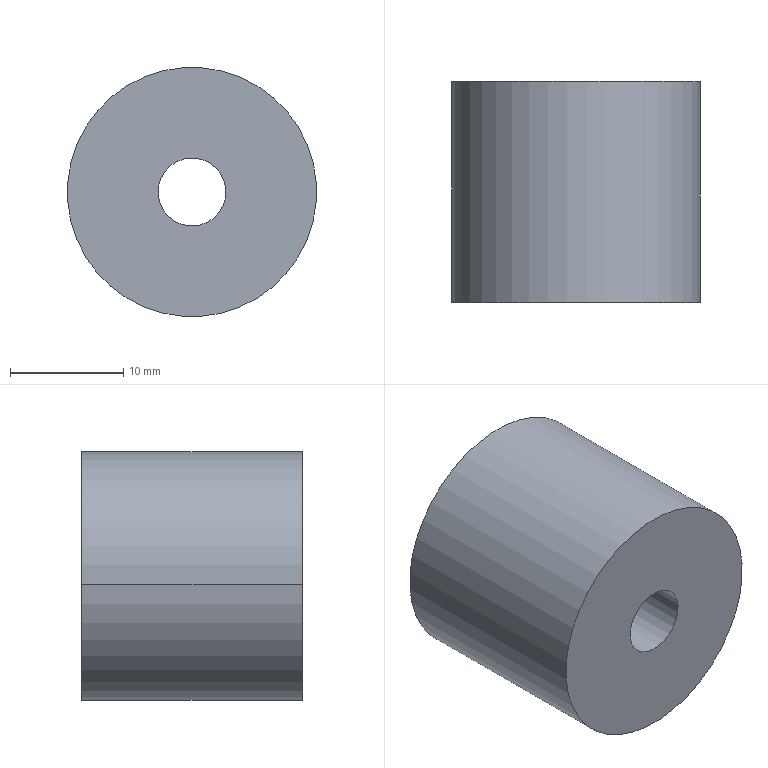Component | SolidWorks | RotaryCylinderSupportPost-1 | 1 solid | 6 faces | box 22 x 19.5 x 22 mm | volume 6861 mm3 | cylinder 4 | plane 2 | commonest cylinder face diameters 6 x2 22 x2
build123d program:
from build123d import *

# Parameters (mm, degrees)
SKETCH2_R           = 11
SKETCH2_R_2         = 3
BOSS_EXTRUDE1_DEPTH = 19.5


with BuildPart() as part:
    # Sketch2 → Boss-Extrude1 (new body)
    with BuildSketch(Plane.XY):
        with Locations((213.487, -329.579)):
            Circle(SKETCH2_R)
        with Locations((213.487, -329.579)):
            Circle(SKETCH2_R_2, mode=Mode.SUBTRACT)
    extrude(amount=BOSS_EXTRUDE1_DEPTH)


solid = part.part

# Placed as in the assembly
solid = solid.moved(Location((-565.183, -108.151, 657.296), (90, 0, 0)))
STEP:
#1=CARTESIAN_POINT('',(-13.964,-4.258,12.894));
#2=VERTEX_POINT('',#1);
#3=CARTESIAN_POINT('',(-13.728,-4.258,12.911));
#4=VERTEX_POINT('',#3);
#5=CARTESIAN_POINT('',(-13.846,-4.258,12.902));
#6=DIRECTION('',(0.,1.,0.));
#7=DIRECTION('',(0.9975,-0.,0.07018));
#8=AXIS2_PLACEMENT_3D('',#5,#6,#7);
#9=CIRCLE('',#8,0.1181);
#10=EDGE_CURVE('',#2,#4,#9,.T.);
#11=ORIENTED_EDGE('',*,*,#10,.T.);
#12=CARTESIAN_POINT('',(-13.728,-5.026,12.911));
#13=VERTEX_POINT('',#12);
#14=CARTESIAN_POINT('',(-13.728,-4.258,12.911));
#15=DIRECTION('',(-0.,-1.,-0.));
#16=VECTOR('',#15,39.37);
#17=LINE('',#14,#16);
#18=EDGE_CURVE('',#4,#13,#17,.T.);
#19=ORIENTED_EDGE('',*,*,#18,.T.);
#20=CARTESIAN_POINT('',(-13.964,-5.026,12.894));
#21=VERTEX_POINT('',#20);
#22=CARTESIAN_POINT('',(-13.846,-5.026,12.902));
#23=DIRECTION('',(0.,1.,0.));
#24=DIRECTION('',(0.9975,0.,0.07018));
#25=AXIS2_PLACEMENT_3D('',#22,#23,#24);
#26=CIRCLE('',#25,0.1181);
#27=EDGE_CURVE('',#21,#13,#26,.T.);
#28=ORIENTED_EDGE('',*,*,#27,.F.);
#29=CARTESIAN_POINT('',(-13.964,-4.258,12.894));
#30=DIRECTION('',(-0.,-1.,-0.));
#31=VECTOR('',#30,39.37);
#32=LINE('',#29,#31);
#33=EDGE_CURVE('',#2,#21,#32,.T.);
#34=ORIENTED_EDGE('',*,*,#33,.F.);
#35=EDGE_LOOP('',(#11,#19,#28,#34));
#36=FACE_OUTER_BOUND('',#35,.T.);
#37=CARTESIAN_POINT('',(-13.846,-4.258,12.902));
#38=DIRECTION('',(-0.,-1.,-0.));
#39=DIRECTION('',(-0.9975,0.,-0.07018));
#40=AXIS2_PLACEMENT_3D('',#37,#38,#39);
#41=CYLINDRICAL_SURFACE('',#40,0.1181);
#42=ADVANCED_FACE('',(#36),#41,.F.);
#43=CARTESIAN_POINT('',(-13.414,-4.258,12.933));
#44=VERTEX_POINT('',#43);
#45=CARTESIAN_POINT('',(-14.278,-4.258,12.872));
#46=VERTEX_POINT('',#45);
#47=CARTESIAN_POINT('',(-13.846,-4.258,12.902));
#48=DIRECTION('',(0.,1.,0.));
#49=DIRECTION('',(0.9975,-0.,0.07018));
#50=AXIS2_PLACEMENT_3D('',#47,#48,#49);
#51=CIRCLE('',#50,0.4331);
#52=EDGE_CURVE('',#44,#46,#51,.T.);
#53=ORIENTED_EDGE('',*,*,#52,.F.);
#54=CARTESIAN_POINT('',(-13.414,-5.026,12.933));
#55=VERTEX_POINT('',#54);
#56=CARTESIAN_POINT('',(-13.414,-4.258,12.933));
#57=DIRECTION('',(-0.,-1.,-0.));
#58=VECTOR('',#57,39.37);
#59=LINE('',#56,#58);
#60=EDGE_CURVE('',#44,#55,#59,.T.);
#61=ORIENTED_EDGE('',*,*,#60,.T.);
#62=CARTESIAN_POINT('',(-14.278,-5.026,12.872));
#63=VERTEX_POINT('',#62);
#64=CARTESIAN_POINT('',(-13.846,-5.026,12.902));
#65=DIRECTION('',(0.,1.,0.));
#66=DIRECTION('',(0.9975,-0.,0.07018));
#67=AXIS2_PLACEMENT_3D('',#64,#65,#66);
#68=CIRCLE('',#67,0.4331);
#69=EDGE_CURVE('',#55,#63,#68,.T.);
#70=ORIENTED_EDGE('',*,*,#69,.T.);
#71=CARTESIAN_POINT('',(-14.278,-4.258,12.872));
#72=DIRECTION('',(-0.,-1.,-0.));
#73=VECTOR('',#72,39.37);
#74=LINE('',#71,#73);
#75=EDGE_CURVE('',#46,#63,#74,.T.);
#76=ORIENTED_EDGE('',*,*,#75,.F.);
#77=EDGE_LOOP('',(#53,#61,#70,#76));
#78=FACE_OUTER_BOUND('',#77,.T.);
#79=CARTESIAN_POINT('',(-13.846,-4.258,12.902));
#80=DIRECTION('',(-0.,-1.,-0.));
#81=DIRECTION('',(-0.9975,0.,-0.07018));
#82=AXIS2_PLACEMENT_3D('',#79,#80,#81);
#83=CYLINDRICAL_SURFACE('',#82,0.4331);
#84=ADVANCED_FACE('',(#78),#83,.T.);
#85=CARTESIAN_POINT('',(-13.846,-4.258,12.902));
#86=DIRECTION('',(0.,1.,0.));
#87=DIRECTION('',(0.9975,-0.,0.07018));
#88=AXIS2_PLACEMENT_3D('',#85,#86,#87);
#89=CIRCLE('',#88,0.4331);
#90=EDGE_CURVE('',#46,#44,#89,.T.);
#91=ORIENTED_EDGE('',*,*,#90,.T.);
#92=ORIENTED_EDGE('',*,*,#52,.T.);
#93=EDGE_LOOP('',(#91,#92));
#94=FACE_OUTER_BOUND('',#93,.T.);
#95=ORIENTED_EDGE('',*,*,#10,.F.);
#96=CARTESIAN_POINT('',(-13.846,-4.258,12.902));
#97=DIRECTION('',(0.,1.,0.));
#98=DIRECTION('',(0.9975,-0.,0.07018));
#99=AXIS2_PLACEMENT_3D('',#96,#97,#98);
#100=CIRCLE('',#99,0.1181);
#101=EDGE_CURVE('',#4,#2,#100,.T.);
#102=ORIENTED_EDGE('',*,*,#101,.F.);
#103=EDGE_LOOP('',(#95,#102));
#104=FACE_BOUND('',#103,.T.);
#105=CARTESIAN_POINT('',(-13.846,-4.258,12.902));
#106=DIRECTION('',(0.,1.,0.));
#107=DIRECTION('',(0.9975,-0.,0.07018));
#108=AXIS2_PLACEMENT_3D('',#105,#106,#107);
#109=PLANE('',#108);
#110=ADVANCED_FACE('',(#94,#104),#109,.T.);
#111=CARTESIAN_POINT('',(-13.846,-5.026,12.902));
#112=DIRECTION('',(0.,1.,0.));
#113=DIRECTION('',(0.9975,-0.,0.07018));
#114=AXIS2_PLACEMENT_3D('',#111,#112,#113);
#115=CIRCLE('',#114,0.4331);
#116=EDGE_CURVE('',#63,#55,#115,.T.);
#117=ORIENTED_EDGE('',*,*,#116,.F.);
#118=ORIENTED_EDGE('',*,*,#69,.F.);
#119=EDGE_LOOP('',(#117,#118));
#120=FACE_OUTER_BOUND('',#119,.T.);
#121=ORIENTED_EDGE('',*,*,#27,.T.);
#122=CARTESIAN_POINT('',(-13.846,-5.026,12.902));
#123=DIRECTION('',(0.,1.,0.));
#124=DIRECTION('',(0.9975,0.,0.07018));
#125=AXIS2_PLACEMENT_3D('',#122,#123,#124);
#126=CIRCLE('',#125,0.1181);
#127=EDGE_CURVE('',#13,#21,#126,.T.);
#128=ORIENTED_EDGE('',*,*,#127,.T.);
#129=EDGE_LOOP('',(#121,#128));
#130=FACE_BOUND('',#129,.T.);
#131=CARTESIAN_POINT('',(-13.846,-5.026,12.902));
#132=DIRECTION('',(0.,1.,0.));
#133=DIRECTION('',(0.9975,-0.,0.07018));
#134=AXIS2_PLACEMENT_3D('',#131,#132,#133);
#135=PLANE('',#134);
#136=ADVANCED_FACE('',(#120,#130),#135,.F.);
#137=ORIENTED_EDGE('',*,*,#60,.F.);
#138=ORIENTED_EDGE('',*,*,#90,.F.);
#139=ORIENTED_EDGE('',*,*,#75,.T.);
#140=ORIENTED_EDGE('',*,*,#116,.T.);
#141=EDGE_LOOP('',(#137,#138,#139,#140));
#142=FACE_OUTER_BOUND('',#141,.T.);
#143=CARTESIAN_POINT('',(-13.846,-4.258,12.902));
#144=DIRECTION('',(-0.,-1.,-0.));
#145=DIRECTION('',(-0.9975,0.,-0.07018));
#146=AXIS2_PLACEMENT_3D('',#143,#144,#145);
#147=CYLINDRICAL_SURFACE('',#146,0.4331);
#148=ADVANCED_FACE('',(#142),#147,.T.);
#149=ORIENTED_EDGE('',*,*,#18,.F.);
#150=ORIENTED_EDGE('',*,*,#101,.T.);
#151=ORIENTED_EDGE('',*,*,#33,.T.);
#152=ORIENTED_EDGE('',*,*,#127,.F.);
#153=EDGE_LOOP('',(#149,#150,#151,#152));
#154=FACE_OUTER_BOUND('',#153,.T.);
#155=CARTESIAN_POINT('',(-13.846,-4.258,12.902));
#156=DIRECTION('',(-0.,-1.,-0.));
#157=DIRECTION('',(-0.9975,0.,-0.07018));
#158=AXIS2_PLACEMENT_3D('',#155,#156,#157);
#159=CYLINDRICAL_SURFACE('',#158,0.1181);
#160=ADVANCED_FACE('',(#154),#159,.F.);
#161=CLOSED_SHELL('',(#42,#84,#110,#136,#148,#160));
#162=MANIFOLD_SOLID_BREP('',#161);
#163=CARTESIAN_POINT('',(0.,0.,0.));
#164=DIRECTION('',(0.,0.,1.));
#165=DIRECTION('',(1.,0.,0.));
#166=AXIS2_PLACEMENT_3D('',#163,#164,#165);
#167=(LENGTH_UNIT()NAMED_UNIT(*)SI_UNIT($,.METRE.));
#168=LENGTH_MEASURE_WITH_UNIT(LENGTH_MEASURE(0.0254),#167);
#169=DIMENSIONAL_EXPONENTS(1.,0.,0.,0.,0.,0.,0.);
#170=(CONVERSION_BASED_UNIT('',#168)LENGTH_UNIT()NAMED_UNIT(#169));
#171=UNCERTAINTY_MEASURE_WITH_UNIT(LENGTH_MEASURE(0.00001),#170,'','');
#172=(NAMED_UNIT(*)PLANE_ANGLE_UNIT()SI_UNIT($,.RADIAN.));
#173=(NAMED_UNIT(*)SI_UNIT($,.STERADIAN.)SOLID_ANGLE_UNIT());
#174=(GEOMETRIC_REPRESENTATION_CONTEXT(3)GLOBAL_UNCERTAINTY_ASSIGNED_CONTEXT((#171))GLOBAL_UNIT_ASSIGNED_CONTEXT((#170,#172,#173))REPRESENTATION_CONTEXT('',''));
#175=ADVANCED_BREP_SHAPE_REPRESENTATION('',(#162,#166),#174);
#176=COLOUR_RGB('',0.7922,0.8196,0.9333);
#177=FILL_AREA_STYLE_COLOUR('',#176);
#178=FILL_AREA_STYLE('',(#177));
#179=SURFACE_STYLE_FILL_AREA(#178);
#180=SURFACE_SIDE_STYLE('',(#179));
#181=SURFACE_STYLE_USAGE(.BOTH.,#180);
#182=PRESENTATION_STYLE_ASSIGNMENT((#181));
#183=STYLED_ITEM('',(#182),#162);
#184=PRESENTATION_LAYER_ASSIGNMENT('','',(#183));
#185=(LENGTH_UNIT()NAMED_UNIT(*)SI_UNIT($,.METRE.));
#186=LENGTH_MEASURE_WITH_UNIT(LENGTH_MEASURE(0.0254),#185);
#187=DIMENSIONAL_EXPONENTS(1.,0.,0.,0.,0.,0.,0.);
#188=(CONVERSION_BASED_UNIT('',#186)LENGTH_UNIT()NAMED_UNIT(#187));
#189=UNCERTAINTY_MEASURE_WITH_UNIT(LENGTH_MEASURE(0.00001),#188,'','');
#190=(NAMED_UNIT(*)PLANE_ANGLE_UNIT()SI_UNIT($,.RADIAN.));
#191=(NAMED_UNIT(*)SI_UNIT($,.STERADIAN.)SOLID_ANGLE_UNIT());
#192=(GEOMETRIC_REPRESENTATION_CONTEXT(3)GLOBAL_UNCERTAINTY_ASSIGNED_CONTEXT((#189))GLOBAL_UNIT_ASSIGNED_CONTEXT((#188,#190,#191))REPRESENTATION_CONTEXT('',''));
#193=MECHANICAL_DESIGN_GEOMETRIC_PRESENTATION_REPRESENTATION('',(#183),#192);